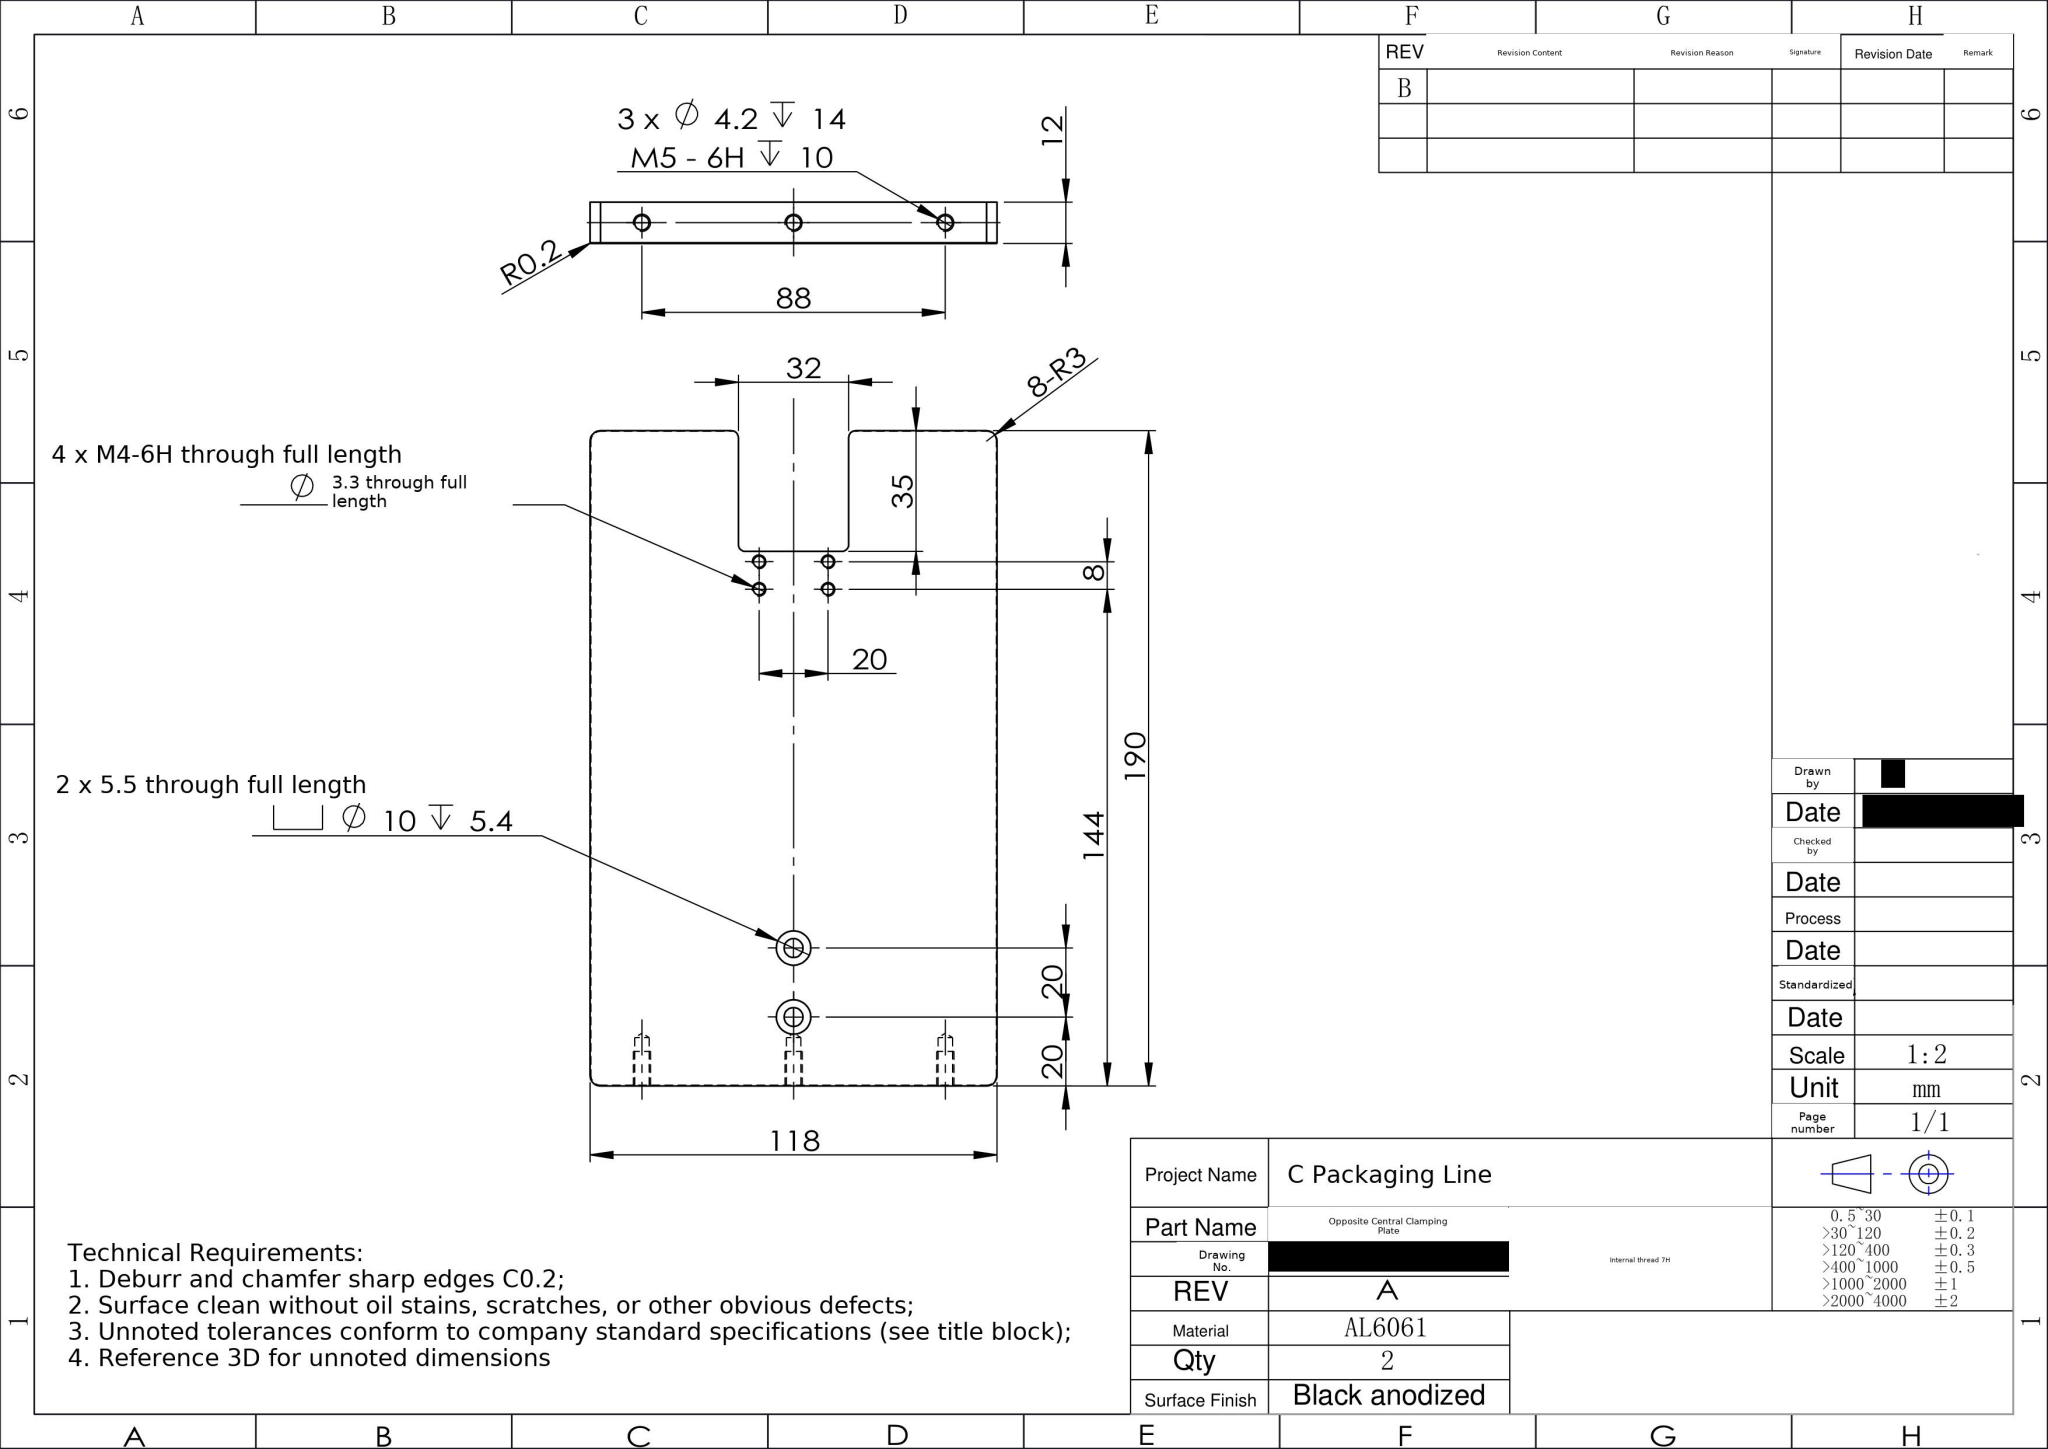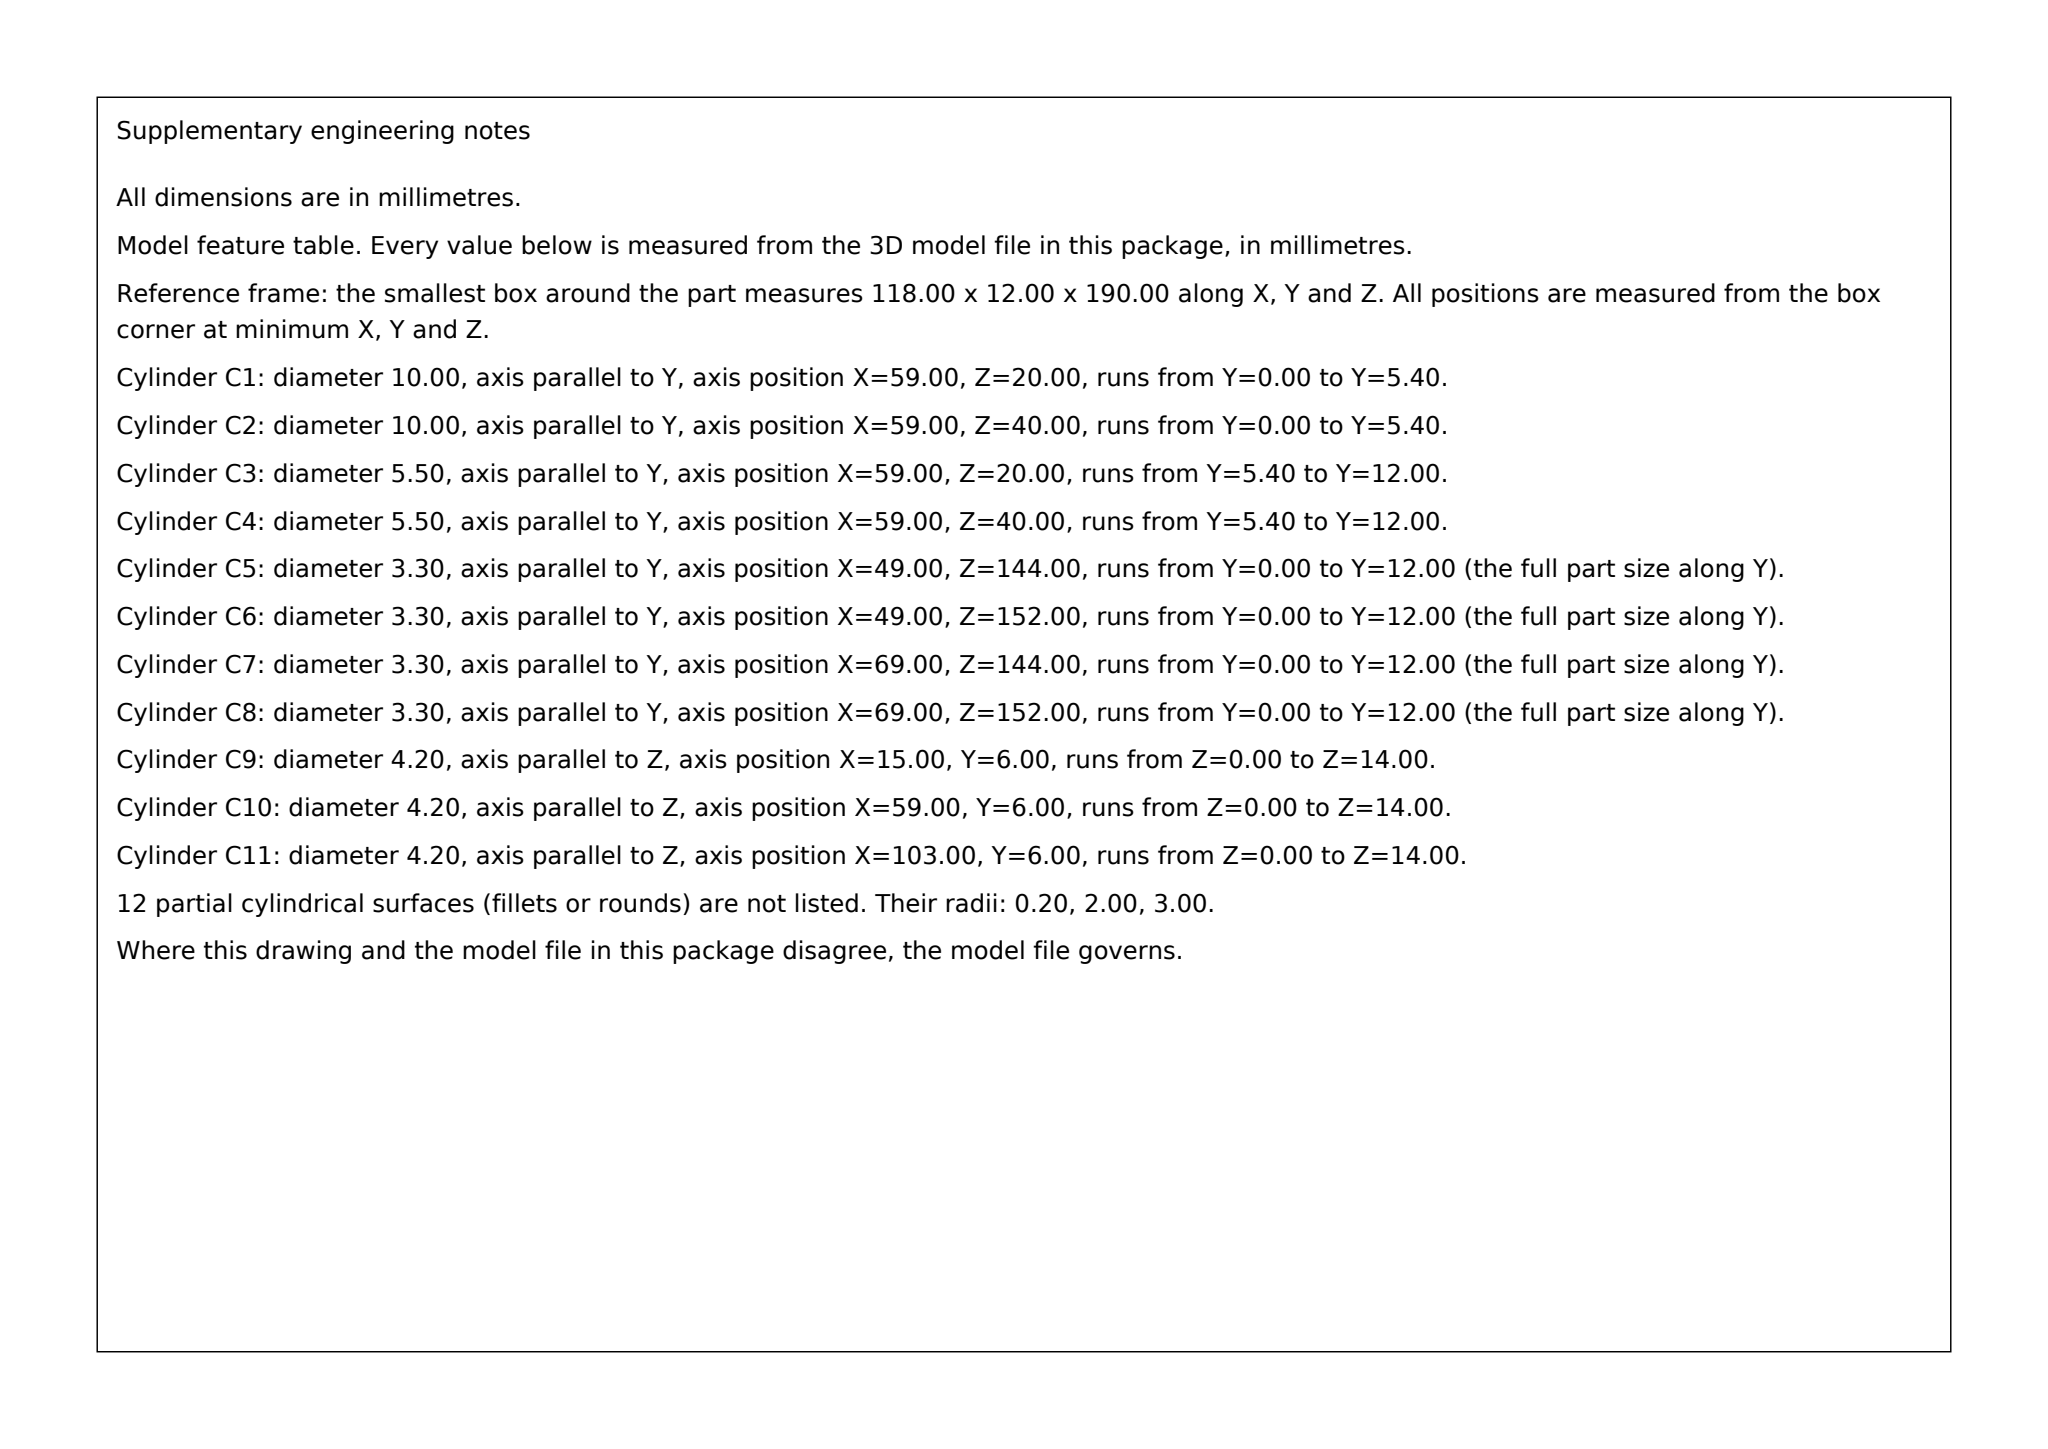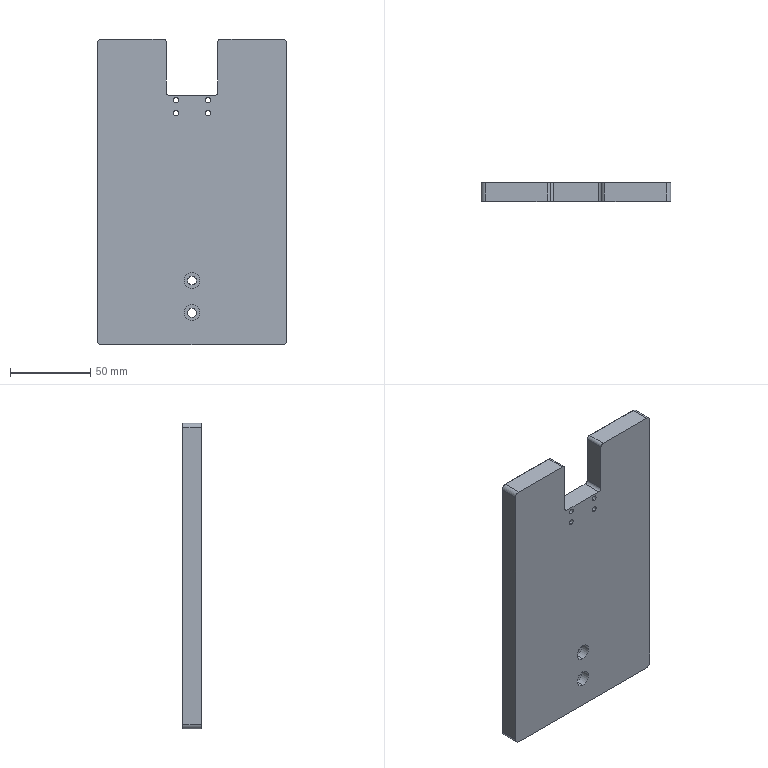Part | SolidWorks | mm | 1 solid | 57 faces | box 118 x 12 x 190 mm | volume 253331 mm3 | cylinder 35 | plane 12 | cone 6 | torus 4 | commonest cylinder face diameters 3.3 x8 4.2 x6 0.4 x5 10 x4 5.5 x4 6 x4 4 x4